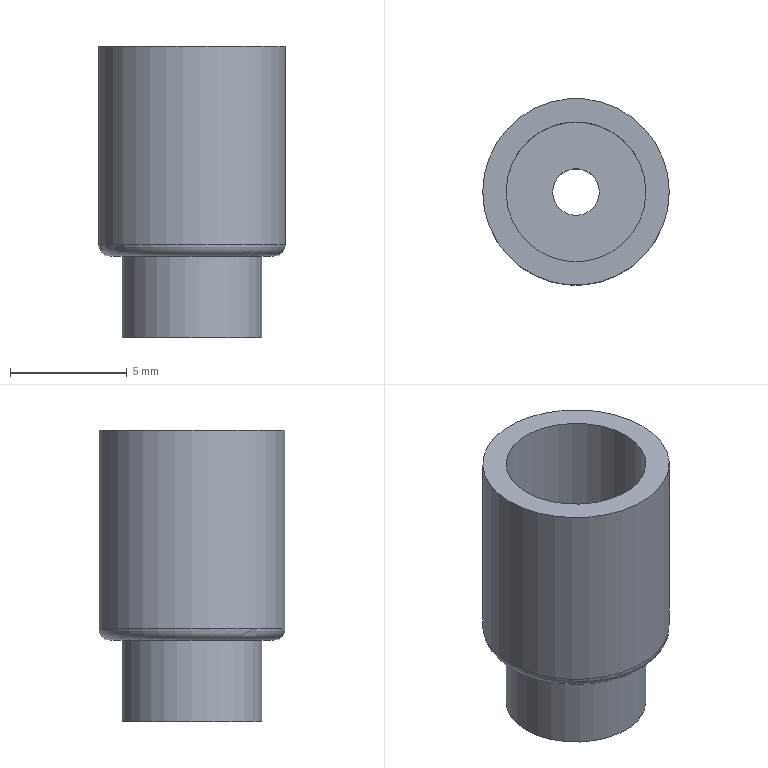Component | NX | VENT_PLUG_2 | 1 solid | 9 faces | box 8 x 8 x 12.5 mm | volume 310 mm3 | plane 4 | cylinder 4 | torus 1 | commonest cylinder face diameters 6 x2 8 x1 2 x1
STEP:
#1=CARTESIAN_POINT('',(0.,0.,0.));
#2=DIRECTION('',(0.,0.,1.));
#3=DIRECTION('',(1.,0.,0.));
#4=AXIS2_PLACEMENT_3D('',#1,#2,#3);
#5=CARTESIAN_POINT('',(-1.,40.,39.));
#6=VERTEX_POINT('',#5);
#7=CARTESIAN_POINT('',(1.,40.,39.));
#8=VERTEX_POINT('',#7);
#9=CARTESIAN_POINT('',(0.,40.,39.));
#10=DIRECTION('',(0.,0.,-1.));
#11=DIRECTION('',(-1.,0.,0.));
#12=AXIS2_PLACEMENT_3D('',#9,#10,#11);
#13=CIRCLE('',#12,1.);
#14=CARTESIAN_POINT('',(0.,40.,39.));
#15=DIRECTION('',(0.,0.,-1.));
#16=DIRECTION('',(-1.,0.,0.));
#17=AXIS2_PLACEMENT_3D('',#14,#15,#16);
#18=PLANE('',#17);
#19=CARTESIAN_POINT('',(0.,0.));
#20=DIRECTION('',(1.,0.));
#21=AXIS2_PLACEMENT_2D('',#19,#20);
#22=CIRCLE('',#21,1.);
#23=(GEOMETRIC_REPRESENTATION_CONTEXT(2)PARAMETRIC_REPRESENTATION_CONTEXT()REPRESENTATION_CONTEXT('',''));
#24=DEFINITIONAL_REPRESENTATION('',(#22),#23);
#25=PCURVE('',#18,#24);
#26=CARTESIAN_POINT('',(0.,40.,35.5));
#27=DIRECTION('',(0.,0.,1.));
#28=DIRECTION('',(1.,0.,0.));
#29=AXIS2_PLACEMENT_3D('',#26,#27,#28);
#30=CYLINDRICAL_SURFACE('',#29,1.);
#31=CARTESIAN_POINT('',(3.142,3.5));
#32=DIRECTION('',(-1.,0.));
#33=VECTOR('',#32,1.);
#34=LINE('',#31,#33);
#35=(GEOMETRIC_REPRESENTATION_CONTEXT(2)PARAMETRIC_REPRESENTATION_CONTEXT()REPRESENTATION_CONTEXT('',''));
#36=DEFINITIONAL_REPRESENTATION('',(#34),#35);
#37=PCURVE('',#30,#36);
#38=SURFACE_CURVE('',#13,(#25,#37),.PCURVE_S1.);
#39=EDGE_CURVE('',#6,#8,#38,.T.);
#40=ORIENTED_EDGE('',*,*,#39,.F.);
#41=CARTESIAN_POINT('',(0.,40.,39.));
#42=DIRECTION('',(0.,0.,-1.));
#43=DIRECTION('',(-1.,0.,0.));
#44=AXIS2_PLACEMENT_3D('',#41,#42,#43);
#45=CIRCLE('',#44,1.);
#46=CARTESIAN_POINT('',(0.,0.));
#47=DIRECTION('',(1.,0.));
#48=AXIS2_PLACEMENT_2D('',#46,#47);
#49=CIRCLE('',#48,1.);
#50=(GEOMETRIC_REPRESENTATION_CONTEXT(2)PARAMETRIC_REPRESENTATION_CONTEXT()REPRESENTATION_CONTEXT('',''));
#51=DEFINITIONAL_REPRESENTATION('',(#49),#50);
#52=PCURVE('',#18,#51);
#53=CARTESIAN_POINT('',(9.425,3.5));
#54=DIRECTION('',(-1.,0.));
#55=VECTOR('',#54,1.);
#56=LINE('',#53,#55);
#57=(GEOMETRIC_REPRESENTATION_CONTEXT(2)PARAMETRIC_REPRESENTATION_CONTEXT()REPRESENTATION_CONTEXT('',''));
#58=DEFINITIONAL_REPRESENTATION('',(#56),#57);
#59=PCURVE('',#30,#58);
#60=SURFACE_CURVE('',#45,(#52,#59),.PCURVE_S1.);
#61=EDGE_CURVE('',#8,#6,#60,.T.);
#62=ORIENTED_EDGE('',*,*,#61,.F.);
#63=EDGE_LOOP('',(#40,#62));
#64=FACE_BOUND('',#63,.T.);
#65=CARTESIAN_POINT('',(3.,40.,39.));
#66=VERTEX_POINT('',#65);
#67=CARTESIAN_POINT('',(0.,40.,39.));
#68=DIRECTION('',(0.,0.,1.));
#69=DIRECTION('',(1.,0.,0.));
#70=AXIS2_PLACEMENT_3D('',#67,#68,#69);
#71=CIRCLE('',#70,3.);
#72=CARTESIAN_POINT('',(-3.,0.));
#73=CARTESIAN_POINT('',(-3.,5.196));
#74=CARTESIAN_POINT('',(1.5,2.598));
#75=CARTESIAN_POINT('',(6.,0.));
#76=CARTESIAN_POINT('',(1.5,-2.598));
#77=CARTESIAN_POINT('',(-3.,-5.196));
#78=CARTESIAN_POINT('',(-3.,0.));
#79=(BOUNDED_CURVE()B_SPLINE_CURVE(2,(#72,#73,#74,#75,#76,#77,#78),.UNSPECIFIED.,.T.,.F.)B_SPLINE_CURVE_WITH_KNOTS((1,2,2,2,2,1),(-2.094,0.,2.094,4.189,6.283,8.378),.UNSPECIFIED.)CURVE()GEOMETRIC_REPRESENTATION_ITEM()RATIONAL_B_SPLINE_CURVE((1.,0.5,1.,0.5,1.,0.5,1.))REPRESENTATION_ITEM(''));
#80=(GEOMETRIC_REPRESENTATION_CONTEXT(2)PARAMETRIC_REPRESENTATION_CONTEXT()REPRESENTATION_CONTEXT('',''));
#81=DEFINITIONAL_REPRESENTATION('',(#79),#80);
#82=PCURVE('',#18,#81);
#83=CARTESIAN_POINT('',(0.,40.,39.));
#84=DIRECTION('',(0.,0.,1.));
#85=DIRECTION('',(1.,0.,0.));
#86=AXIS2_PLACEMENT_3D('',#83,#84,#85);
#87=CYLINDRICAL_SURFACE('',#86,3.);
#88=CARTESIAN_POINT('',(0.,0.));
#89=DIRECTION('',(1.,0.));
#90=VECTOR('',#89,1.);
#91=LINE('',#88,#90);
#92=(GEOMETRIC_REPRESENTATION_CONTEXT(2)PARAMETRIC_REPRESENTATION_CONTEXT()REPRESENTATION_CONTEXT('',''));
#93=DEFINITIONAL_REPRESENTATION('',(#91),#92);
#94=PCURVE('',#87,#93);
#95=SURFACE_CURVE('',#71,(#82,#94),.PCURVE_S1.);
#96=EDGE_CURVE('',#66,#66,#95,.T.);
#97=ORIENTED_EDGE('',*,*,#96,.F.);
#98=EDGE_LOOP('',(#97));
#99=FACE_BOUND('',#98,.T.);
#100=ADVANCED_FACE('',(#64,#99),#18,.T.);
#101=CARTESIAN_POINT('',(3.,40.,42.5));
#102=VERTEX_POINT('',#101);
#103=CARTESIAN_POINT('',(0.,40.,42.5));
#104=DIRECTION('',(0.,0.,-1.));
#105=DIRECTION('',(1.,0.,0.));
#106=AXIS2_PLACEMENT_3D('',#103,#104,#105);
#107=CIRCLE('',#106,3.);
#108=CARTESIAN_POINT('',(6.283,3.5));
#109=DIRECTION('',(-1.,0.));
#110=VECTOR('',#109,1.);
#111=LINE('',#108,#110);
#112=(GEOMETRIC_REPRESENTATION_CONTEXT(2)PARAMETRIC_REPRESENTATION_CONTEXT()REPRESENTATION_CONTEXT('',''));
#113=DEFINITIONAL_REPRESENTATION('',(#111),#112);
#114=PCURVE('',#87,#113);
#115=CARTESIAN_POINT('',(0.,40.,42.5));
#116=DIRECTION('',(0.,0.,-1.));
#117=DIRECTION('',(-1.,0.,0.));
#118=AXIS2_PLACEMENT_3D('',#115,#116,#117);
#119=PLANE('',#118);
#120=CARTESIAN_POINT('',(-0.,0.));
#121=DIRECTION('',(-1.,0.));
#122=AXIS2_PLACEMENT_2D('',#120,#121);
#123=CIRCLE('',#122,3.);
#124=(GEOMETRIC_REPRESENTATION_CONTEXT(2)PARAMETRIC_REPRESENTATION_CONTEXT()REPRESENTATION_CONTEXT('',''));
#125=DEFINITIONAL_REPRESENTATION('',(#123),#124);
#126=PCURVE('',#119,#125);
#127=SURFACE_CURVE('',#107,(#114,#126),.PCURVE_S1.);
#128=EDGE_CURVE('',#102,#102,#127,.T.);
#129=ORIENTED_EDGE('',*,*,#128,.T.);
#130=CARTESIAN_POINT('',(3.,40.,39.));
#131=CARTESIAN_POINT('',(3.,40.,42.5));
#132=B_SPLINE_CURVE_WITH_KNOTS('',1,(#130,#131),.UNSPECIFIED.,.F.,.F.,(2,2),(0.,3.5),.PIECEWISE_BEZIER_KNOTS.);
#133=CARTESIAN_POINT('',(0.,0.));
#134=DIRECTION('',(0.,1.));
#135=VECTOR('',#134,1.);
#136=LINE('',#133,#135);
#137=(GEOMETRIC_REPRESENTATION_CONTEXT(2)PARAMETRIC_REPRESENTATION_CONTEXT()REPRESENTATION_CONTEXT('',''));
#138=DEFINITIONAL_REPRESENTATION('',(#136),#137);
#139=PCURVE('',#87,#138);
#140=CARTESIAN_POINT('',(6.283,0.));
#141=DIRECTION('',(0.,1.));
#142=VECTOR('',#141,1.);
#143=LINE('',#140,#142);
#144=(GEOMETRIC_REPRESENTATION_CONTEXT(2)PARAMETRIC_REPRESENTATION_CONTEXT()REPRESENTATION_CONTEXT('',''));
#145=DEFINITIONAL_REPRESENTATION('',(#143),#144);
#146=PCURVE('',#87,#145);
#147=SEAM_CURVE('',#132,(#139,#146),.PCURVE_S1.);
#148=EDGE_CURVE('',#66,#102,#147,.T.);
#149=ORIENTED_EDGE('',*,*,#148,.F.);
#150=ORIENTED_EDGE('',*,*,#96,.T.);
#151=ORIENTED_EDGE('',*,*,#148,.T.);
#152=EDGE_LOOP('',(#129,#149,#150,#151));
#153=FACE_BOUND('',#152,.T.);
#154=ADVANCED_FACE('',(#153),#87,.T.);
#155=CARTESIAN_POINT('',(3.,40.,51.5));
#156=VERTEX_POINT('',#155);
#157=CARTESIAN_POINT('',(0.,40.,51.5));
#158=DIRECTION('',(0.,0.,1.));
#159=DIRECTION('',(1.,0.,0.));
#160=AXIS2_PLACEMENT_3D('',#157,#158,#159);
#161=CIRCLE('',#160,3.);
#162=CARTESIAN_POINT('',(0.,40.,51.5));
#163=DIRECTION('',(0.,0.,1.));
#164=DIRECTION('',(1.,0.,0.));
#165=AXIS2_PLACEMENT_3D('',#162,#163,#164);
#166=PLANE('',#165);
#167=CARTESIAN_POINT('',(0.,0.));
#168=DIRECTION('',(1.,0.));
#169=AXIS2_PLACEMENT_2D('',#167,#168);
#170=CIRCLE('',#169,3.);
#171=(GEOMETRIC_REPRESENTATION_CONTEXT(2)PARAMETRIC_REPRESENTATION_CONTEXT()REPRESENTATION_CONTEXT('',''));
#172=DEFINITIONAL_REPRESENTATION('',(#170),#171);
#173=PCURVE('',#166,#172);
#174=CARTESIAN_POINT('',(0.,40.,43.5));
#175=DIRECTION('',(0.,0.,1.));
#176=DIRECTION('',(1.,0.,0.));
#177=AXIS2_PLACEMENT_3D('',#174,#175,#176);
#178=CYLINDRICAL_SURFACE('',#177,3.);
#179=CARTESIAN_POINT('',(0.,8.));
#180=DIRECTION('',(1.,0.));
#181=VECTOR('',#180,1.);
#182=LINE('',#179,#181);
#183=(GEOMETRIC_REPRESENTATION_CONTEXT(2)PARAMETRIC_REPRESENTATION_CONTEXT()REPRESENTATION_CONTEXT('',''));
#184=DEFINITIONAL_REPRESENTATION('',(#182),#183);
#185=PCURVE('',#178,#184);
#186=SURFACE_CURVE('',#161,(#173,#185),.PCURVE_S1.);
#187=EDGE_CURVE('',#156,#156,#186,.T.);
#188=ORIENTED_EDGE('',*,*,#187,.F.);
#189=EDGE_LOOP('',(#188));
#190=FACE_BOUND('',#189,.T.);
#191=CARTESIAN_POINT('',(4.,40.,51.5));
#192=VERTEX_POINT('',#191);
#193=CARTESIAN_POINT('',(0.,40.,51.5));
#194=DIRECTION('',(0.,0.,1.));
#195=DIRECTION('',(1.,0.,0.));
#196=AXIS2_PLACEMENT_3D('',#193,#194,#195);
#197=CIRCLE('',#196,4.);
#198=CARTESIAN_POINT('',(0.,0.));
#199=DIRECTION('',(1.,0.));
#200=AXIS2_PLACEMENT_2D('',#198,#199);
#201=CIRCLE('',#200,4.);
#202=(GEOMETRIC_REPRESENTATION_CONTEXT(2)PARAMETRIC_REPRESENTATION_CONTEXT()REPRESENTATION_CONTEXT('',''));
#203=DEFINITIONAL_REPRESENTATION('',(#201),#202);
#204=PCURVE('',#166,#203);
#205=CARTESIAN_POINT('',(0.,40.,42.5));
#206=DIRECTION('',(0.,0.,1.));
#207=DIRECTION('',(1.,0.,0.));
#208=AXIS2_PLACEMENT_3D('',#205,#206,#207);
#209=CYLINDRICAL_SURFACE('',#208,4.);
#210=CARTESIAN_POINT('',(0.,9.));
#211=DIRECTION('',(1.,0.));
#212=VECTOR('',#211,1.);
#213=LINE('',#210,#212);
#214=(GEOMETRIC_REPRESENTATION_CONTEXT(2)PARAMETRIC_REPRESENTATION_CONTEXT()REPRESENTATION_CONTEXT('',''));
#215=DEFINITIONAL_REPRESENTATION('',(#213),#214);
#216=PCURVE('',#209,#215);
#217=SURFACE_CURVE('',#197,(#204,#216),.PCURVE_S1.);
#218=EDGE_CURVE('',#192,#192,#217,.T.);
#219=ORIENTED_EDGE('',*,*,#218,.T.);
#220=EDGE_LOOP('',(#219));
#221=FACE_BOUND('',#220,.T.);
#222=ADVANCED_FACE('',(#190,#221),#166,.T.);
#223=CARTESIAN_POINT('',(-3.5,40.,42.5));
#224=VERTEX_POINT('',#223);
#225=CARTESIAN_POINT('',(0.,40.,42.5));
#226=DIRECTION('',(0.,0.,-1.));
#227=DIRECTION('',(-1.,0.,0.));
#228=AXIS2_PLACEMENT_3D('',#225,#226,#227);
#229=CIRCLE('',#228,3.5);
#230=CARTESIAN_POINT('',(0.,0.));
#231=DIRECTION('',(1.,0.));
#232=AXIS2_PLACEMENT_2D('',#230,#231);
#233=CIRCLE('',#232,3.5);
#234=(GEOMETRIC_REPRESENTATION_CONTEXT(2)PARAMETRIC_REPRESENTATION_CONTEXT()REPRESENTATION_CONTEXT('',''));
#235=DEFINITIONAL_REPRESENTATION('',(#233),#234);
#236=PCURVE('',#119,#235);
#237=CARTESIAN_POINT('',(0.,40.,43.));
#238=DIRECTION('',(0.,0.,-1.));
#239=DIRECTION('',(-1.,0.,0.));
#240=AXIS2_PLACEMENT_3D('',#237,#238,#239);
#241=TOROIDAL_SURFACE('',#240,3.5,0.5);
#242=CARTESIAN_POINT('',(0.,7.854));
#243=DIRECTION('',(1.,0.));
#244=VECTOR('',#243,1.);
#245=LINE('',#242,#244);
#246=(GEOMETRIC_REPRESENTATION_CONTEXT(2)PARAMETRIC_REPRESENTATION_CONTEXT()REPRESENTATION_CONTEXT('',''));
#247=DEFINITIONAL_REPRESENTATION('',(#245),#246);
#248=PCURVE('',#241,#247);
#249=SURFACE_CURVE('',#229,(#236,#248),.PCURVE_S1.);
#250=EDGE_CURVE('',#224,#224,#249,.T.);
#251=ORIENTED_EDGE('',*,*,#250,.T.);
#252=EDGE_LOOP('',(#251));
#253=FACE_BOUND('',#252,.T.);
#254=ORIENTED_EDGE('',*,*,#128,.F.);
#255=EDGE_LOOP('',(#254));
#256=FACE_BOUND('',#255,.T.);
#257=ADVANCED_FACE('',(#253,#256),#119,.T.);
#258=CARTESIAN_POINT('',(-4.,40.,43.));
#259=VERTEX_POINT('',#258);
#260=CARTESIAN_POINT('',(4.,40.,43.));
#261=VERTEX_POINT('',#260);
#262=CARTESIAN_POINT('',(0.,40.,43.));
#263=DIRECTION('',(0.,0.,1.));
#264=DIRECTION('',(-1.,0.,0.));
#265=AXIS2_PLACEMENT_3D('',#262,#263,#264);
#266=CIRCLE('',#265,4.);
#267=CARTESIAN_POINT('',(3.142,0.5));
#268=DIRECTION('',(1.,0.));
#269=VECTOR('',#268,1.);
#270=LINE('',#267,#269);
#271=(GEOMETRIC_REPRESENTATION_CONTEXT(2)PARAMETRIC_REPRESENTATION_CONTEXT()REPRESENTATION_CONTEXT('',''));
#272=DEFINITIONAL_REPRESENTATION('',(#270),#271);
#273=PCURVE('',#209,#272);
#274=CARTESIAN_POINT('',(6.283,6.283));
#275=DIRECTION('',(-1.,0.));
#276=VECTOR('',#275,1.);
#277=LINE('',#274,#276);
#278=(GEOMETRIC_REPRESENTATION_CONTEXT(2)PARAMETRIC_REPRESENTATION_CONTEXT()REPRESENTATION_CONTEXT('',''));
#279=DEFINITIONAL_REPRESENTATION('',(#277),#278);
#280=PCURVE('',#241,#279);
#281=SURFACE_CURVE('',#266,(#273,#280),.PCURVE_S1.);
#282=EDGE_CURVE('',#259,#261,#281,.T.);
#283=ORIENTED_EDGE('',*,*,#282,.T.);
#284=CARTESIAN_POINT('',(4.,40.,43.));
#285=CARTESIAN_POINT('',(4.,40.,51.5));
#286=B_SPLINE_CURVE_WITH_KNOTS('',1,(#284,#285),.UNSPECIFIED.,.F.,.F.,(2,2),(0.5,9.),.PIECEWISE_BEZIER_KNOTS.);
#287=CARTESIAN_POINT('',(6.283,0.));
#288=DIRECTION('',(0.,1.));
#289=VECTOR('',#288,1.);
#290=LINE('',#287,#289);
#291=(GEOMETRIC_REPRESENTATION_CONTEXT(2)PARAMETRIC_REPRESENTATION_CONTEXT()REPRESENTATION_CONTEXT('',''));
#292=DEFINITIONAL_REPRESENTATION('',(#290),#291);
#293=PCURVE('',#209,#292);
#294=CARTESIAN_POINT('',(0.,0.));
#295=DIRECTION('',(0.,1.));
#296=VECTOR('',#295,1.);
#297=LINE('',#294,#296);
#298=(GEOMETRIC_REPRESENTATION_CONTEXT(2)PARAMETRIC_REPRESENTATION_CONTEXT()REPRESENTATION_CONTEXT('',''));
#299=DEFINITIONAL_REPRESENTATION('',(#297),#298);
#300=PCURVE('',#209,#299);
#301=SEAM_CURVE('',#286,(#293,#300),.PCURVE_S1.);
#302=EDGE_CURVE('',#261,#192,#301,.T.);
#303=ORIENTED_EDGE('',*,*,#302,.T.);
#304=ORIENTED_EDGE('',*,*,#218,.F.);
#305=ORIENTED_EDGE('',*,*,#302,.F.);
#306=CARTESIAN_POINT('',(0.,40.,43.));
#307=DIRECTION('',(0.,0.,1.));
#308=DIRECTION('',(-1.,0.,0.));
#309=AXIS2_PLACEMENT_3D('',#306,#307,#308);
#310=CIRCLE('',#309,4.);
#311=CARTESIAN_POINT('',(-3.142,0.5));
#312=DIRECTION('',(1.,0.));
#313=VECTOR('',#312,1.);
#314=LINE('',#311,#313);
#315=(GEOMETRIC_REPRESENTATION_CONTEXT(2)PARAMETRIC_REPRESENTATION_CONTEXT()REPRESENTATION_CONTEXT('',''));
#316=DEFINITIONAL_REPRESENTATION('',(#314),#315);
#317=PCURVE('',#209,#316);
#318=CARTESIAN_POINT('',(6.283,6.283));
#319=DIRECTION('',(-1.,0.));
#320=VECTOR('',#319,1.);
#321=LINE('',#318,#320);
#322=(GEOMETRIC_REPRESENTATION_CONTEXT(2)PARAMETRIC_REPRESENTATION_CONTEXT()REPRESENTATION_CONTEXT('',''));
#323=DEFINITIONAL_REPRESENTATION('',(#321),#322);
#324=PCURVE('',#241,#323);
#325=SURFACE_CURVE('',#310,(#317,#324),.PCURVE_S1.);
#326=EDGE_CURVE('',#261,#259,#325,.T.);
#327=ORIENTED_EDGE('',*,*,#326,.T.);
#328=EDGE_LOOP('',(#283,#303,#304,#305,#327));
#329=FACE_BOUND('',#328,.T.);
#330=ADVANCED_FACE('',(#329),#209,.T.);
#331=CARTESIAN_POINT('',(3.,40.,43.5));
#332=VERTEX_POINT('',#331);
#333=CARTESIAN_POINT('',(0.,40.,43.5));
#334=DIRECTION('',(0.,0.,-1.));
#335=DIRECTION('',(1.,0.,0.));
#336=AXIS2_PLACEMENT_3D('',#333,#334,#335);
#337=CIRCLE('',#336,3.);
#338=CARTESIAN_POINT('',(6.283,0.));
#339=DIRECTION('',(-1.,0.));
#340=VECTOR('',#339,1.);
#341=LINE('',#338,#340);
#342=(GEOMETRIC_REPRESENTATION_CONTEXT(2)PARAMETRIC_REPRESENTATION_CONTEXT()REPRESENTATION_CONTEXT('',''));
#343=DEFINITIONAL_REPRESENTATION('',(#341),#342);
#344=PCURVE('',#178,#343);
#345=CARTESIAN_POINT('',(0.,40.,43.5));
#346=DIRECTION('',(0.,0.,1.));
#347=DIRECTION('',(1.,0.,0.));
#348=AXIS2_PLACEMENT_3D('',#345,#346,#347);
#349=PLANE('',#348);
#350=CARTESIAN_POINT('',(3.,0.));
#351=CARTESIAN_POINT('',(3.,-5.196));
#352=CARTESIAN_POINT('',(-1.5,-2.598));
#353=CARTESIAN_POINT('',(-6.,-0.));
#354=CARTESIAN_POINT('',(-1.5,2.598));
#355=CARTESIAN_POINT('',(3.,5.196));
#356=CARTESIAN_POINT('',(3.,0.));
#357=(BOUNDED_CURVE()B_SPLINE_CURVE(2,(#350,#351,#352,#353,#354,#355,#356),.UNSPECIFIED.,.T.,.F.)B_SPLINE_CURVE_WITH_KNOTS((1,2,2,2,2,1),(-2.094,0.,2.094,4.189,6.283,8.378),.UNSPECIFIED.)CURVE()GEOMETRIC_REPRESENTATION_ITEM()RATIONAL_B_SPLINE_CURVE((1.,0.5,1.,0.5,1.,0.5,1.))REPRESENTATION_ITEM(''));
#358=(GEOMETRIC_REPRESENTATION_CONTEXT(2)PARAMETRIC_REPRESENTATION_CONTEXT()REPRESENTATION_CONTEXT('',''));
#359=DEFINITIONAL_REPRESENTATION('',(#357),#358);
#360=PCURVE('',#349,#359);
#361=SURFACE_CURVE('',#337,(#344,#360),.PCURVE_S1.);
#362=EDGE_CURVE('',#332,#332,#361,.T.);
#363=ORIENTED_EDGE('',*,*,#362,.F.);
#364=CARTESIAN_POINT('',(3.,40.,43.5));
#365=CARTESIAN_POINT('',(3.,40.,51.5));
#366=B_SPLINE_CURVE_WITH_KNOTS('',1,(#364,#365),.UNSPECIFIED.,.F.,.F.,(2,2),(0.,8.),.PIECEWISE_BEZIER_KNOTS.);
#367=CARTESIAN_POINT('',(6.283,0.));
#368=DIRECTION('',(0.,1.));
#369=VECTOR('',#368,1.);
#370=LINE('',#367,#369);
#371=(GEOMETRIC_REPRESENTATION_CONTEXT(2)PARAMETRIC_REPRESENTATION_CONTEXT()REPRESENTATION_CONTEXT('',''));
#372=DEFINITIONAL_REPRESENTATION('',(#370),#371);
#373=PCURVE('',#178,#372);
#374=CARTESIAN_POINT('',(0.,0.));
#375=DIRECTION('',(0.,1.));
#376=VECTOR('',#375,1.);
#377=LINE('',#374,#376);
#378=(GEOMETRIC_REPRESENTATION_CONTEXT(2)PARAMETRIC_REPRESENTATION_CONTEXT()REPRESENTATION_CONTEXT('',''));
#379=DEFINITIONAL_REPRESENTATION('',(#377),#378);
#380=PCURVE('',#178,#379);
#381=SEAM_CURVE('',#366,(#373,#380),.PCURVE_S1.);
#382=EDGE_CURVE('',#332,#156,#381,.T.);
#383=ORIENTED_EDGE('',*,*,#382,.T.);
#384=ORIENTED_EDGE('',*,*,#187,.F.);
#385=ORIENTED_EDGE('',*,*,#382,.F.);
#386=EDGE_LOOP('',(#363,#383,#384,#385));
#387=FACE_BOUND('',#386,.F.);
#388=ADVANCED_FACE('',(#387),#178,.F.);
#389=CARTESIAN_POINT('',(1.,40.,43.5));
#390=VERTEX_POINT('',#389);
#391=CARTESIAN_POINT('',(0.,40.,43.5));
#392=DIRECTION('',(0.,0.,1.));
#393=DIRECTION('',(1.,0.,0.));
#394=AXIS2_PLACEMENT_3D('',#391,#392,#393);
#395=CIRCLE('',#394,1.);
#396=CARTESIAN_POINT('',(-0.,0.));
#397=DIRECTION('',(1.,0.));
#398=AXIS2_PLACEMENT_2D('',#396,#397);
#399=CIRCLE('',#398,1.);
#400=(GEOMETRIC_REPRESENTATION_CONTEXT(2)PARAMETRIC_REPRESENTATION_CONTEXT()REPRESENTATION_CONTEXT('',''));
#401=DEFINITIONAL_REPRESENTATION('',(#399),#400);
#402=PCURVE('',#349,#401);
#403=CARTESIAN_POINT('',(0.,8.));
#404=DIRECTION('',(1.,0.));
#405=VECTOR('',#404,1.);
#406=LINE('',#403,#405);
#407=(GEOMETRIC_REPRESENTATION_CONTEXT(2)PARAMETRIC_REPRESENTATION_CONTEXT()REPRESENTATION_CONTEXT('',''));
#408=DEFINITIONAL_REPRESENTATION('',(#406),#407);
#409=PCURVE('',#30,#408);
#410=SURFACE_CURVE('',#395,(#402,#409),.PCURVE_S1.);
#411=EDGE_CURVE('',#390,#390,#410,.T.);
#412=ORIENTED_EDGE('',*,*,#411,.F.);
#413=EDGE_LOOP('',(#412));
#414=FACE_BOUND('',#413,.T.);
#415=ORIENTED_EDGE('',*,*,#362,.F.);
#416=EDGE_LOOP('',(#415));
#417=FACE_BOUND('',#416,.T.);
#418=ADVANCED_FACE('',(#414,#417),#349,.T.);
#419=ORIENTED_EDGE('',*,*,#250,.F.);
#420=CARTESIAN_POINT('',(-4.,40.,43.));
#421=CARTESIAN_POINT('',(-4.,40.,42.866));
#422=CARTESIAN_POINT('',(-3.957,40.,42.736));
#423=CARTESIAN_POINT('',(-3.876,40.,42.624));
#424=CARTESIAN_POINT('',(-3.764,40.,42.543));
#425=CARTESIAN_POINT('',(-3.634,40.,42.5));
#426=CARTESIAN_POINT('',(-3.5,40.,42.5));
#427=(BOUNDED_CURVE()B_SPLINE_CURVE(6,(#420,#421,#422,#423,#424,#425,#426),.UNSPECIFIED.,.F.,.F.)B_SPLINE_CURVE_WITH_KNOTS((7,7),(0.,1.571),.PIECEWISE_BEZIER_KNOTS.)CURVE()GEOMETRIC_REPRESENTATION_ITEM()RATIONAL_B_SPLINE_CURVE((1.031,1.01,0.9979,0.994,0.9979,1.01,1.031))REPRESENTATION_ITEM(''));
#428=CARTESIAN_POINT('',(0.,6.283));
#429=DIRECTION('',(0.,1.));
#430=VECTOR('',#429,1.);
#431=LINE('',#428,#430);
#432=(GEOMETRIC_REPRESENTATION_CONTEXT(2)PARAMETRIC_REPRESENTATION_CONTEXT()REPRESENTATION_CONTEXT('',''));
#433=DEFINITIONAL_REPRESENTATION('',(#431),#432);
#434=PCURVE('',#241,#433);
#435=CARTESIAN_POINT('',(6.283,6.283));
#436=DIRECTION('',(0.,1.));
#437=VECTOR('',#436,1.);
#438=LINE('',#435,#437);
#439=(GEOMETRIC_REPRESENTATION_CONTEXT(2)PARAMETRIC_REPRESENTATION_CONTEXT()REPRESENTATION_CONTEXT('',''));
#440=DEFINITIONAL_REPRESENTATION('',(#438),#439);
#441=PCURVE('',#241,#440);
#442=SEAM_CURVE('',#427,(#434,#441),.PCURVE_S1.);
#443=EDGE_CURVE('',#259,#224,#442,.T.);
#444=ORIENTED_EDGE('',*,*,#443,.F.);
#445=ORIENTED_EDGE('',*,*,#326,.F.);
#446=ORIENTED_EDGE('',*,*,#282,.F.);
#447=ORIENTED_EDGE('',*,*,#443,.T.);
#448=EDGE_LOOP('',(#419,#444,#445,#446,#447));
#449=FACE_BOUND('',#448,.T.);
#450=ADVANCED_FACE('',(#449),#241,.T.);
#451=ORIENTED_EDGE('',*,*,#61,.F.);
#452=CARTESIAN_POINT('',(1.,40.,39.));
#453=CARTESIAN_POINT('',(1.,40.,43.5));
#454=B_SPLINE_CURVE_WITH_KNOTS('',1,(#452,#453),.UNSPECIFIED.,.F.,.F.,(2,2),(3.5,8.),.PIECEWISE_BEZIER_KNOTS.);
#455=CARTESIAN_POINT('',(6.283,0.));
#456=DIRECTION('',(0.,1.));
#457=VECTOR('',#456,1.);
#458=LINE('',#455,#457);
#459=(GEOMETRIC_REPRESENTATION_CONTEXT(2)PARAMETRIC_REPRESENTATION_CONTEXT()REPRESENTATION_CONTEXT('',''));
#460=DEFINITIONAL_REPRESENTATION('',(#458),#459);
#461=PCURVE('',#30,#460);
#462=CARTESIAN_POINT('',(0.,0.));
#463=DIRECTION('',(0.,1.));
#464=VECTOR('',#463,1.);
#465=LINE('',#462,#464);
#466=(GEOMETRIC_REPRESENTATION_CONTEXT(2)PARAMETRIC_REPRESENTATION_CONTEXT()REPRESENTATION_CONTEXT('',''));
#467=DEFINITIONAL_REPRESENTATION('',(#465),#466);
#468=PCURVE('',#30,#467);
#469=SEAM_CURVE('',#454,(#461,#468),.PCURVE_S1.);
#470=EDGE_CURVE('',#8,#390,#469,.T.);
#471=ORIENTED_EDGE('',*,*,#470,.T.);
#472=ORIENTED_EDGE('',*,*,#411,.F.);
#473=ORIENTED_EDGE('',*,*,#470,.F.);
#474=ORIENTED_EDGE('',*,*,#39,.F.);
#475=EDGE_LOOP('',(#451,#471,#472,#473,#474));
#476=FACE_BOUND('',#475,.F.);
#477=ADVANCED_FACE('',(#476),#30,.F.);
#478=CLOSED_SHELL('',(#100,#154,#222,#257,#330,#388,#418,#450,#477));
#479=MANIFOLD_SOLID_BREP('',#478);
#480=(LENGTH_UNIT()NAMED_UNIT(*)SI_UNIT(.MILLI.,.METRE.));
#481=UNCERTAINTY_MEASURE_WITH_UNIT(LENGTH_MEASURE(0.00001),#480,'','');
#482=(NAMED_UNIT(*)PLANE_ANGLE_UNIT()SI_UNIT($,.RADIAN.));
#483=(NAMED_UNIT(*)SI_UNIT($,.STERADIAN.)SOLID_ANGLE_UNIT());
#484=(GEOMETRIC_REPRESENTATION_CONTEXT(3)GLOBAL_UNCERTAINTY_ASSIGNED_CONTEXT((#481))GLOBAL_UNIT_ASSIGNED_CONTEXT((#480,#482,#483))REPRESENTATION_CONTEXT('',''));
#485=ADVANCED_BREP_SHAPE_REPRESENTATION('',(#4,#479),#484);